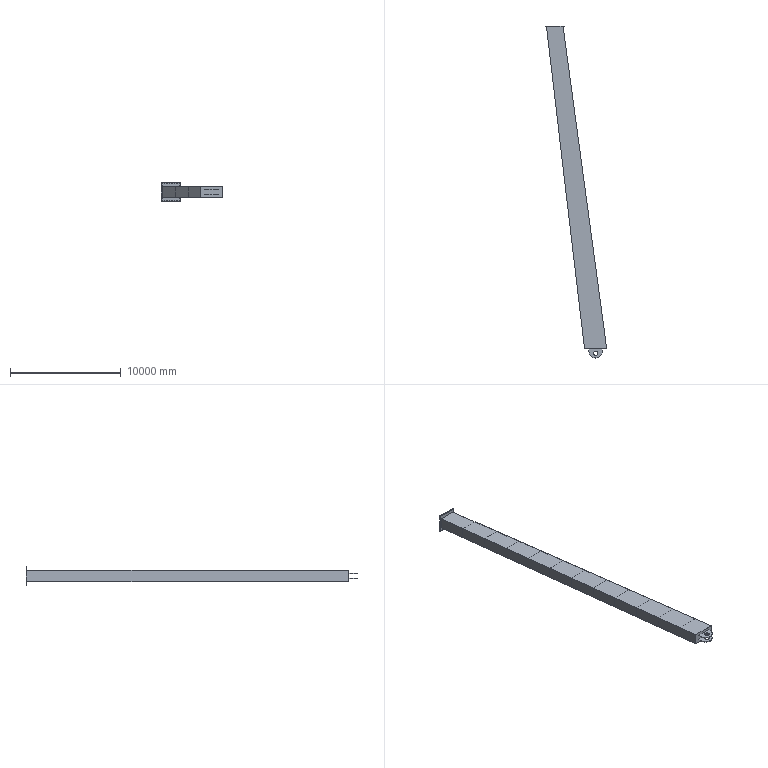Component | SolidWorks | FlexibleLegGenuine-2 | 1 solid | 181 faces | volume 7566927915 mm3 | plane 93 | cylinder 64 | spline 24 | commonest cylinder face diameters 40 x56 400 x4 1200 x4